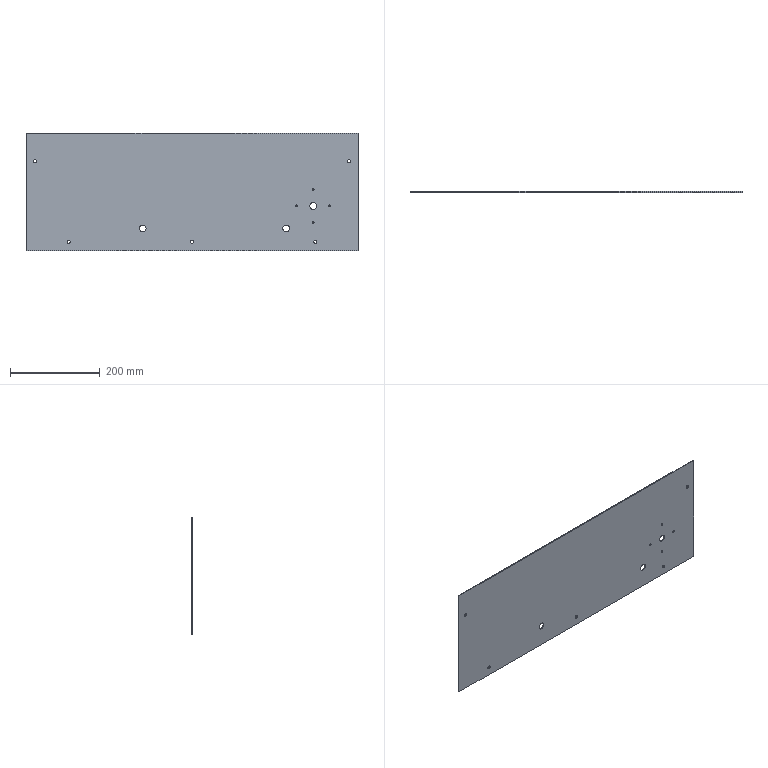Component | SolidWorks | 30-42A-1 | 1 solid | 30 faces | box 740 x 2 x 262 mm | volume 386204 mm3 | cylinder 24 | plane 6 | commonest cylinder face diameters 7 x10 4.2 x8 15 x6
build123d program:
from build123d import *

# Parameters (mm, degrees)
SKETCH1_W             = 740
SKETCH1_H             = 262
EXTRUDE1_DEPTH        = 2
SKETCH2_R             = 7.5
CUT_EXTRUDE1_DEPTH    = 10
SKETCH3_R             = 3.5
CUT_EXTRUDE2_DEPTH    = 10
M5_TAPPED_HOLE1_D     = 4.2
M5_TAPPED_HOLE1_DEPTH = 12.4
M5_TAPPED_HOLE1_TIP   = 1.262


with BuildPart() as part:
    # Sketch1 → Extrude1 (new body)
    with BuildSketch(Plane.XY):
        Rectangle(SKETCH1_W, SKETCH1_H)
    extrude(amount=EXTRUDE1_DEPTH)

    # Sketch2 → Cut-Extrude1 (cut)
    with BuildSketch(Plane.XY.offset(2)):
        with Locations((270, 31)):
            Circle(SKETCH2_R)
        with Locations((210, 81)):
            Circle(SKETCH2_R)
        with Locations((-110, 81)):
            Circle(SKETCH2_R)
    extrude(amount=-CUT_EXTRUDE1_DEPTH, mode=Mode.SUBTRACT)

    # Sketch3 → Cut-Extrude2 (cut)
    with BuildSketch(Plane.XY.offset(2)):
        with Locations((-275, 111)):
            Circle(SKETCH3_R)
        with Locations((0, 111)):
            Circle(SKETCH3_R)
        with Locations((-350, -69)):
            Circle(SKETCH3_R)
        with Locations((350, -69)):
            Circle(SKETCH3_R)
        with Locations((275, 111)):
            Circle(SKETCH3_R)
    extrude(amount=-CUT_EXTRUDE2_DEPTH, mode=Mode.SUBTRACT)

    # M5 Tapped Hole1
    with Locations(Plane.XY.offset(2)):
        with Locations((270, 67.5), (233.5, 31), (270, -5.5), (306.5, 31)):
            Hole(M5_TAPPED_HOLE1_D / 2, depth=M5_TAPPED_HOLE1_DEPTH)
            with Locations((0, 0, -(M5_TAPPED_HOLE1_DEPTH + M5_TAPPED_HOLE1_TIP / 2))):  # 118° drill point
                Cone(0, M5_TAPPED_HOLE1_D / 2, M5_TAPPED_HOLE1_TIP, mode=Mode.SUBTRACT)


solid = part.part

# Placed as in the assembly
solid = solid.moved(Location((-77.43, 712.155, -959), (-90, 0, 0)))
STEP:
#1=COLOUR_RGB('',0.7922,0.8196,0.9333);
#2=FILL_AREA_STYLE_COLOUR('',#1);
#3=FILL_AREA_STYLE('',(#2));
#4=SURFACE_STYLE_FILL_AREA(#3);
#5=SURFACE_SIDE_STYLE('',(#4));
#6=SURFACE_STYLE_USAGE(.BOTH.,#5);
#7=PRESENTATION_STYLE_ASSIGNMENT((#6));
#8=CARTESIAN_POINT('',(7.499,28.038,-40.413));
#9=VERTEX_POINT('',#8);
#10=CARTESIAN_POINT('',(7.664,28.038,-40.413));
#11=VERTEX_POINT('',#10);
#12=CARTESIAN_POINT('',(7.582,28.038,-40.413));
#13=DIRECTION('',(0.,1.,0.));
#14=DIRECTION('',(1.,0.,0.));
#15=AXIS2_PLACEMENT_3D('',#12,#13,#14);
#16=CIRCLE('',#15,0.08268);
#17=EDGE_CURVE('',#9,#11,#16,.T.);
#18=ORIENTED_EDGE('',*,*,#17,.F.);
#19=CARTESIAN_POINT('',(7.499,28.116,-40.413));
#20=VERTEX_POINT('',#19);
#21=CARTESIAN_POINT('',(7.499,28.116,-40.413));
#22=DIRECTION('',(0.,1.,0.));
#23=VECTOR('',#22,39.37);
#24=LINE('',#21,#23);
#25=EDGE_CURVE('',#9,#20,#24,.T.);
#26=ORIENTED_EDGE('',*,*,#25,.T.);
#27=CARTESIAN_POINT('',(7.664,28.116,-40.413));
#28=VERTEX_POINT('',#27);
#29=CARTESIAN_POINT('',(7.582,28.116,-40.413));
#30=DIRECTION('',(0.,1.,0.));
#31=DIRECTION('',(1.,0.,0.));
#32=AXIS2_PLACEMENT_3D('',#29,#30,#31);
#33=CIRCLE('',#32,0.08268);
#34=EDGE_CURVE('',#20,#28,#33,.T.);
#35=ORIENTED_EDGE('',*,*,#34,.T.);
#36=CARTESIAN_POINT('',(7.664,28.116,-40.413));
#37=DIRECTION('',(0.,1.,0.));
#38=VECTOR('',#37,39.37);
#39=LINE('',#36,#38);
#40=EDGE_CURVE('',#11,#28,#39,.T.);
#41=ORIENTED_EDGE('',*,*,#40,.F.);
#42=EDGE_LOOP('',(#18,#26,#35,#41));
#43=FACE_OUTER_BOUND('',#42,.T.);
#44=CARTESIAN_POINT('',(7.582,28.116,-40.413));
#45=DIRECTION('',(0.,1.,0.));
#46=DIRECTION('',(1.,0.,0.));
#47=AXIS2_PLACEMENT_3D('',#44,#45,#46);
#48=CYLINDRICAL_SURFACE('',#47,0.08268);
#49=ADVANCED_FACE('',(#43),#48,.F.);
#50=CARTESIAN_POINT('',(6.062,28.038,-38.976));
#51=VERTEX_POINT('',#50);
#52=CARTESIAN_POINT('',(6.227,28.038,-38.976));
#53=VERTEX_POINT('',#52);
#54=CARTESIAN_POINT('',(6.145,28.038,-38.976));
#55=DIRECTION('',(0.,1.,0.));
#56=DIRECTION('',(1.,0.,0.));
#57=AXIS2_PLACEMENT_3D('',#54,#55,#56);
#58=CIRCLE('',#57,0.08268);
#59=EDGE_CURVE('',#51,#53,#58,.T.);
#60=ORIENTED_EDGE('',*,*,#59,.F.);
#61=CARTESIAN_POINT('',(6.062,28.116,-38.976));
#62=VERTEX_POINT('',#61);
#63=CARTESIAN_POINT('',(6.062,28.116,-38.976));
#64=DIRECTION('',(0.,1.,0.));
#65=VECTOR('',#64,39.37);
#66=LINE('',#63,#65);
#67=EDGE_CURVE('',#51,#62,#66,.T.);
#68=ORIENTED_EDGE('',*,*,#67,.T.);
#69=CARTESIAN_POINT('',(6.227,28.116,-38.976));
#70=VERTEX_POINT('',#69);
#71=CARTESIAN_POINT('',(6.145,28.116,-38.976));
#72=DIRECTION('',(0.,1.,0.));
#73=DIRECTION('',(1.,0.,0.));
#74=AXIS2_PLACEMENT_3D('',#71,#72,#73);
#75=CIRCLE('',#74,0.08268);
#76=EDGE_CURVE('',#62,#70,#75,.T.);
#77=ORIENTED_EDGE('',*,*,#76,.T.);
#78=CARTESIAN_POINT('',(6.227,28.116,-38.976));
#79=DIRECTION('',(0.,1.,0.));
#80=VECTOR('',#79,39.37);
#81=LINE('',#78,#80);
#82=EDGE_CURVE('',#53,#70,#81,.T.);
#83=ORIENTED_EDGE('',*,*,#82,.F.);
#84=EDGE_LOOP('',(#60,#68,#77,#83));
#85=FACE_OUTER_BOUND('',#84,.T.);
#86=CARTESIAN_POINT('',(6.145,28.116,-38.976));
#87=DIRECTION('',(0.,1.,0.));
#88=DIRECTION('',(1.,0.,0.));
#89=AXIS2_PLACEMENT_3D('',#86,#87,#88);
#90=CYLINDRICAL_SURFACE('',#89,0.08268);
#91=ADVANCED_FACE('',(#85),#90,.F.);
#92=CARTESIAN_POINT('',(7.499,28.038,-37.539));
#93=VERTEX_POINT('',#92);
#94=CARTESIAN_POINT('',(7.664,28.038,-37.539));
#95=VERTEX_POINT('',#94);
#96=CARTESIAN_POINT('',(7.582,28.038,-37.539));
#97=DIRECTION('',(0.,1.,0.));
#98=DIRECTION('',(1.,0.,0.));
#99=AXIS2_PLACEMENT_3D('',#96,#97,#98);
#100=CIRCLE('',#99,0.08268);
#101=EDGE_CURVE('',#93,#95,#100,.T.);
#102=ORIENTED_EDGE('',*,*,#101,.F.);
#103=CARTESIAN_POINT('',(7.499,28.116,-37.539));
#104=VERTEX_POINT('',#103);
#105=CARTESIAN_POINT('',(7.499,28.116,-37.539));
#106=DIRECTION('',(0.,1.,0.));
#107=VECTOR('',#106,39.37);
#108=LINE('',#105,#107);
#109=EDGE_CURVE('',#93,#104,#108,.T.);
#110=ORIENTED_EDGE('',*,*,#109,.T.);
#111=CARTESIAN_POINT('',(7.664,28.116,-37.539));
#112=VERTEX_POINT('',#111);
#113=CARTESIAN_POINT('',(7.582,28.116,-37.539));
#114=DIRECTION('',(0.,1.,0.));
#115=DIRECTION('',(1.,0.,0.));
#116=AXIS2_PLACEMENT_3D('',#113,#114,#115);
#117=CIRCLE('',#116,0.08268);
#118=EDGE_CURVE('',#104,#112,#117,.T.);
#119=ORIENTED_EDGE('',*,*,#118,.T.);
#120=CARTESIAN_POINT('',(7.664,28.116,-37.539));
#121=DIRECTION('',(0.,1.,0.));
#122=VECTOR('',#121,39.37);
#123=LINE('',#120,#122);
#124=EDGE_CURVE('',#95,#112,#123,.T.);
#125=ORIENTED_EDGE('',*,*,#124,.F.);
#126=EDGE_LOOP('',(#102,#110,#119,#125));
#127=FACE_OUTER_BOUND('',#126,.T.);
#128=CARTESIAN_POINT('',(7.582,28.116,-37.539));
#129=DIRECTION('',(0.,1.,0.));
#130=DIRECTION('',(1.,0.,0.));
#131=AXIS2_PLACEMENT_3D('',#128,#129,#130);
#132=CYLINDRICAL_SURFACE('',#131,0.08268);
#133=ADVANCED_FACE('',(#127),#132,.F.);
#134=CARTESIAN_POINT('',(8.936,28.038,-38.976));
#135=VERTEX_POINT('',#134);
#136=CARTESIAN_POINT('',(9.101,28.038,-38.976));
#137=VERTEX_POINT('',#136);
#138=CARTESIAN_POINT('',(9.019,28.038,-38.976));
#139=DIRECTION('',(0.,1.,0.));
#140=DIRECTION('',(1.,0.,0.));
#141=AXIS2_PLACEMENT_3D('',#138,#139,#140);
#142=CIRCLE('',#141,0.08268);
#143=EDGE_CURVE('',#135,#137,#142,.T.);
#144=ORIENTED_EDGE('',*,*,#143,.F.);
#145=CARTESIAN_POINT('',(8.936,28.116,-38.976));
#146=VERTEX_POINT('',#145);
#147=CARTESIAN_POINT('',(8.936,28.116,-38.976));
#148=DIRECTION('',(0.,1.,0.));
#149=VECTOR('',#148,39.37);
#150=LINE('',#147,#149);
#151=EDGE_CURVE('',#135,#146,#150,.T.);
#152=ORIENTED_EDGE('',*,*,#151,.T.);
#153=CARTESIAN_POINT('',(9.101,28.116,-38.976));
#154=VERTEX_POINT('',#153);
#155=CARTESIAN_POINT('',(9.019,28.116,-38.976));
#156=DIRECTION('',(0.,1.,0.));
#157=DIRECTION('',(1.,0.,0.));
#158=AXIS2_PLACEMENT_3D('',#155,#156,#157);
#159=CIRCLE('',#158,0.08268);
#160=EDGE_CURVE('',#146,#154,#159,.T.);
#161=ORIENTED_EDGE('',*,*,#160,.T.);
#162=CARTESIAN_POINT('',(9.101,28.116,-38.976));
#163=DIRECTION('',(0.,1.,0.));
#164=VECTOR('',#163,39.37);
#165=LINE('',#162,#164);
#166=EDGE_CURVE('',#137,#154,#165,.T.);
#167=ORIENTED_EDGE('',*,*,#166,.F.);
#168=EDGE_LOOP('',(#144,#152,#161,#167));
#169=FACE_OUTER_BOUND('',#168,.T.);
#170=CARTESIAN_POINT('',(9.019,28.116,-38.976));
#171=DIRECTION('',(0.,1.,0.));
#172=DIRECTION('',(1.,0.,0.));
#173=AXIS2_PLACEMENT_3D('',#170,#171,#172);
#174=CYLINDRICAL_SURFACE('',#173,0.08268);
#175=ADVANCED_FACE('',(#169),#174,.F.);
#176=CARTESIAN_POINT('',(7.641,28.038,-42.126));
#177=VERTEX_POINT('',#176);
#178=CARTESIAN_POINT('',(7.916,28.038,-42.126));
#179=VERTEX_POINT('',#178);
#180=CARTESIAN_POINT('',(7.778,28.038,-42.126));
#181=DIRECTION('',(0.,1.,0.));
#182=DIRECTION('',(1.,0.,0.));
#183=AXIS2_PLACEMENT_3D('',#180,#181,#182);
#184=CIRCLE('',#183,0.1378);
#185=EDGE_CURVE('',#177,#179,#184,.T.);
#186=ORIENTED_EDGE('',*,*,#185,.F.);
#187=CARTESIAN_POINT('',(7.641,28.116,-42.126));
#188=VERTEX_POINT('',#187);
#189=CARTESIAN_POINT('',(7.641,27.723,-42.126));
#190=DIRECTION('',(0.,1.,0.));
#191=VECTOR('',#190,39.37);
#192=LINE('',#189,#191);
#193=EDGE_CURVE('',#177,#188,#192,.T.);
#194=ORIENTED_EDGE('',*,*,#193,.T.);
#195=CARTESIAN_POINT('',(7.916,28.116,-42.126));
#196=VERTEX_POINT('',#195);
#197=CARTESIAN_POINT('',(7.778,28.116,-42.126));
#198=DIRECTION('',(0.,1.,0.));
#199=DIRECTION('',(-1.,0.,0.));
#200=AXIS2_PLACEMENT_3D('',#197,#198,#199);
#201=CIRCLE('',#200,0.1378);
#202=EDGE_CURVE('',#188,#196,#201,.T.);
#203=ORIENTED_EDGE('',*,*,#202,.T.);
#204=CARTESIAN_POINT('',(7.916,27.723,-42.126));
#205=DIRECTION('',(0.,1.,0.));
#206=VECTOR('',#205,39.37);
#207=LINE('',#204,#206);
#208=EDGE_CURVE('',#179,#196,#207,.T.);
#209=ORIENTED_EDGE('',*,*,#208,.F.);
#210=EDGE_LOOP('',(#186,#194,#203,#209));
#211=FACE_OUTER_BOUND('',#210,.T.);
#212=CARTESIAN_POINT('',(7.778,27.723,-42.126));
#213=DIRECTION('',(0.,1.,0.));
#214=DIRECTION('',(1.,0.,0.));
#215=AXIS2_PLACEMENT_3D('',#212,#213,#214);
#216=CYLINDRICAL_SURFACE('',#215,0.1378);
#217=ADVANCED_FACE('',(#211),#216,.F.);
#218=CARTESIAN_POINT('',(10.593,28.038,-35.039));
#219=VERTEX_POINT('',#218);
#220=CARTESIAN_POINT('',(10.869,28.038,-35.039));
#221=VERTEX_POINT('',#220);
#222=CARTESIAN_POINT('',(10.731,28.038,-35.039));
#223=DIRECTION('',(0.,1.,0.));
#224=DIRECTION('',(1.,0.,0.));
#225=AXIS2_PLACEMENT_3D('',#222,#223,#224);
#226=CIRCLE('',#225,0.1378);
#227=EDGE_CURVE('',#219,#221,#226,.T.);
#228=ORIENTED_EDGE('',*,*,#227,.F.);
#229=CARTESIAN_POINT('',(10.593,28.116,-35.039));
#230=VERTEX_POINT('',#229);
#231=CARTESIAN_POINT('',(10.593,27.723,-35.039));
#232=DIRECTION('',(0.,1.,0.));
#233=VECTOR('',#232,39.37);
#234=LINE('',#231,#233);
#235=EDGE_CURVE('',#219,#230,#234,.T.);
#236=ORIENTED_EDGE('',*,*,#235,.T.);
#237=CARTESIAN_POINT('',(10.869,28.116,-35.039));
#238=VERTEX_POINT('',#237);
#239=CARTESIAN_POINT('',(10.731,28.116,-35.039));
#240=DIRECTION('',(0.,1.,0.));
#241=DIRECTION('',(-1.,0.,0.));
#242=AXIS2_PLACEMENT_3D('',#239,#240,#241);
#243=CIRCLE('',#242,0.1378);
#244=EDGE_CURVE('',#230,#238,#243,.T.);
#245=ORIENTED_EDGE('',*,*,#244,.T.);
#246=CARTESIAN_POINT('',(10.869,27.723,-35.039));
#247=DIRECTION('',(0.,1.,0.));
#248=VECTOR('',#247,39.37);
#249=LINE('',#246,#248);
#250=EDGE_CURVE('',#221,#238,#249,.T.);
#251=ORIENTED_EDGE('',*,*,#250,.F.);
#252=EDGE_LOOP('',(#228,#236,#245,#251));
#253=FACE_OUTER_BOUND('',#252,.T.);
#254=CARTESIAN_POINT('',(10.731,27.723,-35.039));
#255=DIRECTION('',(0.,1.,0.));
#256=DIRECTION('',(1.,0.,0.));
#257=AXIS2_PLACEMENT_3D('',#254,#255,#256);
#258=CYLINDRICAL_SURFACE('',#257,0.1378);
#259=ADVANCED_FACE('',(#253),#258,.F.);
#260=CARTESIAN_POINT('',(-16.966,28.038,-35.039));
#261=VERTEX_POINT('',#260);
#262=CARTESIAN_POINT('',(-16.69,28.038,-35.039));
#263=VERTEX_POINT('',#262);
#264=CARTESIAN_POINT('',(-16.828,28.038,-35.039));
#265=DIRECTION('',(0.,1.,0.));
#266=DIRECTION('',(1.,0.,0.));
#267=AXIS2_PLACEMENT_3D('',#264,#265,#266);
#268=CIRCLE('',#267,0.1378);
#269=EDGE_CURVE('',#261,#263,#268,.T.);
#270=ORIENTED_EDGE('',*,*,#269,.F.);
#271=CARTESIAN_POINT('',(-16.966,28.116,-35.039));
#272=VERTEX_POINT('',#271);
#273=CARTESIAN_POINT('',(-16.966,27.723,-35.039));
#274=DIRECTION('',(0.,1.,0.));
#275=VECTOR('',#274,39.37);
#276=LINE('',#273,#275);
#277=EDGE_CURVE('',#261,#272,#276,.T.);
#278=ORIENTED_EDGE('',*,*,#277,.T.);
#279=CARTESIAN_POINT('',(-16.69,28.116,-35.039));
#280=VERTEX_POINT('',#279);
#281=CARTESIAN_POINT('',(-16.828,28.116,-35.039));
#282=DIRECTION('',(0.,1.,0.));
#283=DIRECTION('',(1.,0.,0.));
#284=AXIS2_PLACEMENT_3D('',#281,#282,#283);
#285=CIRCLE('',#284,0.1378);
#286=EDGE_CURVE('',#272,#280,#285,.T.);
#287=ORIENTED_EDGE('',*,*,#286,.T.);
#288=CARTESIAN_POINT('',(-16.69,27.723,-35.039));
#289=DIRECTION('',(0.,1.,0.));
#290=VECTOR('',#289,39.37);
#291=LINE('',#288,#290);
#292=EDGE_CURVE('',#263,#280,#291,.T.);
#293=ORIENTED_EDGE('',*,*,#292,.F.);
#294=EDGE_LOOP('',(#270,#278,#287,#293));
#295=FACE_OUTER_BOUND('',#294,.T.);
#296=CARTESIAN_POINT('',(-16.828,27.723,-35.039));
#297=DIRECTION('',(0.,1.,0.));
#298=DIRECTION('',(1.,0.,0.));
#299=AXIS2_PLACEMENT_3D('',#296,#297,#298);
#300=CYLINDRICAL_SURFACE('',#299,0.1378);
#301=ADVANCED_FACE('',(#295),#300,.F.);
#302=CARTESIAN_POINT('',(-3.186,28.038,-42.126));
#303=VERTEX_POINT('',#302);
#304=CARTESIAN_POINT('',(-2.911,28.038,-42.126));
#305=VERTEX_POINT('',#304);
#306=CARTESIAN_POINT('',(-3.048,28.038,-42.126));
#307=DIRECTION('',(0.,1.,0.));
#308=DIRECTION('',(1.,0.,0.));
#309=AXIS2_PLACEMENT_3D('',#306,#307,#308);
#310=CIRCLE('',#309,0.1378);
#311=EDGE_CURVE('',#303,#305,#310,.T.);
#312=ORIENTED_EDGE('',*,*,#311,.F.);
#313=CARTESIAN_POINT('',(-3.186,28.116,-42.126));
#314=VERTEX_POINT('',#313);
#315=CARTESIAN_POINT('',(-3.186,27.723,-42.126));
#316=DIRECTION('',(0.,1.,0.));
#317=VECTOR('',#316,39.37);
#318=LINE('',#315,#317);
#319=EDGE_CURVE('',#303,#314,#318,.T.);
#320=ORIENTED_EDGE('',*,*,#319,.T.);
#321=CARTESIAN_POINT('',(-2.911,28.116,-42.126));
#322=VERTEX_POINT('',#321);
#323=CARTESIAN_POINT('',(-3.048,28.116,-42.126));
#324=DIRECTION('',(0.,1.,0.));
#325=DIRECTION('',(1.,0.,0.));
#326=AXIS2_PLACEMENT_3D('',#323,#324,#325);
#327=CIRCLE('',#326,0.1378);
#328=EDGE_CURVE('',#314,#322,#327,.T.);
#329=ORIENTED_EDGE('',*,*,#328,.T.);
#330=CARTESIAN_POINT('',(-2.911,27.723,-42.126));
#331=DIRECTION('',(0.,1.,0.));
#332=VECTOR('',#331,39.37);
#333=LINE('',#330,#332);
#334=EDGE_CURVE('',#305,#322,#333,.T.);
#335=ORIENTED_EDGE('',*,*,#334,.F.);
#336=EDGE_LOOP('',(#312,#320,#329,#335));
#337=FACE_OUTER_BOUND('',#336,.T.);
#338=CARTESIAN_POINT('',(-3.048,27.723,-42.126));
#339=DIRECTION('',(0.,1.,0.));
#340=DIRECTION('',(1.,0.,0.));
#341=AXIS2_PLACEMENT_3D('',#338,#339,#340);
#342=CYLINDRICAL_SURFACE('',#341,0.1378);
#343=ADVANCED_FACE('',(#337),#342,.F.);
#344=CARTESIAN_POINT('',(-14.013,28.038,-42.126));
#345=VERTEX_POINT('',#344);
#346=CARTESIAN_POINT('',(-13.737,28.038,-42.126));
#347=VERTEX_POINT('',#346);
#348=CARTESIAN_POINT('',(-13.875,28.038,-42.126));
#349=DIRECTION('',(0.,1.,0.));
#350=DIRECTION('',(1.,0.,0.));
#351=AXIS2_PLACEMENT_3D('',#348,#349,#350);
#352=CIRCLE('',#351,0.1378);
#353=EDGE_CURVE('',#345,#347,#352,.T.);
#354=ORIENTED_EDGE('',*,*,#353,.F.);
#355=CARTESIAN_POINT('',(-14.013,28.116,-42.126));
#356=VERTEX_POINT('',#355);
#357=CARTESIAN_POINT('',(-14.013,27.723,-42.126));
#358=DIRECTION('',(0.,1.,0.));
#359=VECTOR('',#358,39.37);
#360=LINE('',#357,#359);
#361=EDGE_CURVE('',#345,#356,#360,.T.);
#362=ORIENTED_EDGE('',*,*,#361,.T.);
#363=CARTESIAN_POINT('',(-13.737,28.116,-42.126));
#364=VERTEX_POINT('',#363);
#365=CARTESIAN_POINT('',(-13.875,28.116,-42.126));
#366=DIRECTION('',(0.,1.,0.));
#367=DIRECTION('',(1.,0.,0.));
#368=AXIS2_PLACEMENT_3D('',#365,#366,#367);
#369=CIRCLE('',#368,0.1378);
#370=EDGE_CURVE('',#356,#364,#369,.T.);
#371=ORIENTED_EDGE('',*,*,#370,.T.);
#372=CARTESIAN_POINT('',(-13.737,27.723,-42.126));
#373=DIRECTION('',(0.,1.,0.));
#374=VECTOR('',#373,39.37);
#375=LINE('',#372,#374);
#376=EDGE_CURVE('',#347,#364,#375,.T.);
#377=ORIENTED_EDGE('',*,*,#376,.F.);
#378=EDGE_LOOP('',(#354,#362,#371,#377));
#379=FACE_OUTER_BOUND('',#378,.T.);
#380=CARTESIAN_POINT('',(-13.875,27.723,-42.126));
#381=DIRECTION('',(0.,1.,0.));
#382=DIRECTION('',(1.,0.,0.));
#383=AXIS2_PLACEMENT_3D('',#380,#381,#382);
#384=CYLINDRICAL_SURFACE('',#383,0.1378);
#385=ADVANCED_FACE('',(#379),#384,.F.);
#386=CARTESIAN_POINT('',(-7.674,28.038,-40.945));
#387=VERTEX_POINT('',#386);
#388=CARTESIAN_POINT('',(-7.084,28.038,-40.945));
#389=VERTEX_POINT('',#388);
#390=CARTESIAN_POINT('',(-7.379,28.038,-40.945));
#391=DIRECTION('',(0.,1.,0.));
#392=DIRECTION('',(1.,0.,0.));
#393=AXIS2_PLACEMENT_3D('',#390,#391,#392);
#394=CIRCLE('',#393,0.2953);
#395=EDGE_CURVE('',#387,#389,#394,.T.);
#396=ORIENTED_EDGE('',*,*,#395,.F.);
#397=CARTESIAN_POINT('',(-7.674,28.116,-40.945));
#398=VERTEX_POINT('',#397);
#399=CARTESIAN_POINT('',(-7.674,27.723,-40.945));
#400=DIRECTION('',(0.,1.,0.));
#401=VECTOR('',#400,39.37);
#402=LINE('',#399,#401);
#403=EDGE_CURVE('',#387,#398,#402,.T.);
#404=ORIENTED_EDGE('',*,*,#403,.T.);
#405=CARTESIAN_POINT('',(-7.084,28.116,-40.945));
#406=VERTEX_POINT('',#405);
#407=CARTESIAN_POINT('',(-7.379,28.116,-40.945));
#408=DIRECTION('',(0.,1.,0.));
#409=DIRECTION('',(1.,0.,0.));
#410=AXIS2_PLACEMENT_3D('',#407,#408,#409);
#411=CIRCLE('',#410,0.2953);
#412=EDGE_CURVE('',#398,#406,#411,.T.);
#413=ORIENTED_EDGE('',*,*,#412,.T.);
#414=CARTESIAN_POINT('',(-7.084,27.723,-40.945));
#415=DIRECTION('',(0.,1.,0.));
#416=VECTOR('',#415,39.37);
#417=LINE('',#414,#416);
#418=EDGE_CURVE('',#389,#406,#417,.T.);
#419=ORIENTED_EDGE('',*,*,#418,.F.);
#420=EDGE_LOOP('',(#396,#404,#413,#419));
#421=FACE_OUTER_BOUND('',#420,.T.);
#422=CARTESIAN_POINT('',(-7.379,27.723,-40.945));
#423=DIRECTION('',(0.,1.,0.));
#424=DIRECTION('',(1.,0.,0.));
#425=AXIS2_PLACEMENT_3D('',#422,#423,#424);
#426=CYLINDRICAL_SURFACE('',#425,0.2953);
#427=ADVANCED_FACE('',(#421),#426,.F.);
#428=CARTESIAN_POINT('',(4.924,28.038,-40.945));
#429=VERTEX_POINT('',#428);
#430=CARTESIAN_POINT('',(5.515,28.038,-40.945));
#431=VERTEX_POINT('',#430);
#432=CARTESIAN_POINT('',(5.219,28.038,-40.945));
#433=DIRECTION('',(0.,1.,0.));
#434=DIRECTION('',(1.,0.,0.));
#435=AXIS2_PLACEMENT_3D('',#432,#433,#434);
#436=CIRCLE('',#435,0.2953);
#437=EDGE_CURVE('',#429,#431,#436,.T.);
#438=ORIENTED_EDGE('',*,*,#437,.F.);
#439=CARTESIAN_POINT('',(4.924,28.116,-40.945));
#440=VERTEX_POINT('',#439);
#441=CARTESIAN_POINT('',(4.924,27.723,-40.945));
#442=DIRECTION('',(0.,1.,0.));
#443=VECTOR('',#442,39.37);
#444=LINE('',#441,#443);
#445=EDGE_CURVE('',#429,#440,#444,.T.);
#446=ORIENTED_EDGE('',*,*,#445,.T.);
#447=CARTESIAN_POINT('',(5.515,28.116,-40.945));
#448=VERTEX_POINT('',#447);
#449=CARTESIAN_POINT('',(5.219,28.116,-40.945));
#450=DIRECTION('',(0.,1.,0.));
#451=DIRECTION('',(1.,0.,0.));
#452=AXIS2_PLACEMENT_3D('',#449,#450,#451);
#453=CIRCLE('',#452,0.2953);
#454=EDGE_CURVE('',#440,#448,#453,.T.);
#455=ORIENTED_EDGE('',*,*,#454,.T.);
#456=CARTESIAN_POINT('',(5.515,27.723,-40.945));
#457=DIRECTION('',(0.,1.,0.));
#458=VECTOR('',#457,39.37);
#459=LINE('',#456,#458);
#460=EDGE_CURVE('',#431,#448,#459,.T.);
#461=ORIENTED_EDGE('',*,*,#460,.F.);
#462=EDGE_LOOP('',(#438,#446,#455,#461));
#463=FACE_OUTER_BOUND('',#462,.T.);
#464=CARTESIAN_POINT('',(5.219,27.723,-40.945));
#465=DIRECTION('',(0.,1.,0.));
#466=DIRECTION('',(1.,0.,0.));
#467=AXIS2_PLACEMENT_3D('',#464,#465,#466);
#468=CYLINDRICAL_SURFACE('',#467,0.2953);
#469=ADVANCED_FACE('',(#463),#468,.F.);
#470=CARTESIAN_POINT('',(7.286,28.038,-38.976));
#471=VERTEX_POINT('',#470);
#472=CARTESIAN_POINT('',(7.877,28.038,-38.976));
#473=VERTEX_POINT('',#472);
#474=CARTESIAN_POINT('',(7.582,28.038,-38.976));
#475=DIRECTION('',(0.,1.,0.));
#476=DIRECTION('',(1.,0.,0.));
#477=AXIS2_PLACEMENT_3D('',#474,#475,#476);
#478=CIRCLE('',#477,0.2953);
#479=EDGE_CURVE('',#471,#473,#478,.T.);
#480=ORIENTED_EDGE('',*,*,#479,.F.);
#481=CARTESIAN_POINT('',(7.286,28.116,-38.976));
#482=VERTEX_POINT('',#481);
#483=CARTESIAN_POINT('',(7.286,27.723,-38.976));
#484=DIRECTION('',(0.,1.,0.));
#485=VECTOR('',#484,39.37);
#486=LINE('',#483,#485);
#487=EDGE_CURVE('',#471,#482,#486,.T.);
#488=ORIENTED_EDGE('',*,*,#487,.T.);
#489=CARTESIAN_POINT('',(7.877,28.116,-38.976));
#490=VERTEX_POINT('',#489);
#491=CARTESIAN_POINT('',(7.582,28.116,-38.976));
#492=DIRECTION('',(0.,1.,0.));
#493=DIRECTION('',(1.,0.,0.));
#494=AXIS2_PLACEMENT_3D('',#491,#492,#493);
#495=CIRCLE('',#494,0.2953);
#496=EDGE_CURVE('',#482,#490,#495,.T.);
#497=ORIENTED_EDGE('',*,*,#496,.T.);
#498=CARTESIAN_POINT('',(7.877,27.723,-38.976));
#499=DIRECTION('',(0.,1.,0.));
#500=VECTOR('',#499,39.37);
#501=LINE('',#498,#500);
#502=EDGE_CURVE('',#473,#490,#501,.T.);
#503=ORIENTED_EDGE('',*,*,#502,.F.);
#504=EDGE_LOOP('',(#480,#488,#497,#503));
#505=FACE_OUTER_BOUND('',#504,.T.);
#506=CARTESIAN_POINT('',(7.582,27.723,-38.976));
#507=DIRECTION('',(0.,1.,0.));
#508=DIRECTION('',(1.,0.,0.));
#509=AXIS2_PLACEMENT_3D('',#506,#507,#508);
#510=CYLINDRICAL_SURFACE('',#509,0.2953);
#511=ADVANCED_FACE('',(#505),#510,.F.);
#512=CARTESIAN_POINT('',(-17.615,28.038,-42.913));
#513=VERTEX_POINT('',#512);
#514=CARTESIAN_POINT('',(-17.615,28.038,-32.598));
#515=VERTEX_POINT('',#514);
#516=CARTESIAN_POINT('',(-17.615,28.038,-42.913));
#517=DIRECTION('',(0.,-0.,1.));
#518=VECTOR('',#517,39.37);
#519=LINE('',#516,#518);
#520=EDGE_CURVE('',#513,#515,#519,.T.);
#521=ORIENTED_EDGE('',*,*,#520,.T.);
#522=CARTESIAN_POINT('',(-17.615,28.116,-32.598));
#523=VERTEX_POINT('',#522);
#524=CARTESIAN_POINT('',(-17.615,28.116,-32.598));
#525=DIRECTION('',(-0.,-1.,-0.));
#526=VECTOR('',#525,39.37);
#527=LINE('',#524,#526);
#528=EDGE_CURVE('',#523,#515,#527,.T.);
#529=ORIENTED_EDGE('',*,*,#528,.F.);
#530=CARTESIAN_POINT('',(-17.615,28.116,-42.913));
#531=VERTEX_POINT('',#530);
#532=CARTESIAN_POINT('',(-17.615,28.116,-42.913));
#533=DIRECTION('',(0.,-0.,1.));
#534=VECTOR('',#533,39.37);
#535=LINE('',#532,#534);
#536=EDGE_CURVE('',#531,#523,#535,.T.);
#537=ORIENTED_EDGE('',*,*,#536,.F.);
#538=CARTESIAN_POINT('',(-17.615,28.116,-42.913));
#539=DIRECTION('',(-0.,-1.,-0.));
#540=VECTOR('',#539,39.37);
#541=LINE('',#538,#540);
#542=EDGE_CURVE('',#531,#513,#541,.T.);
#543=ORIENTED_EDGE('',*,*,#542,.T.);
#544=EDGE_LOOP('',(#521,#529,#537,#543));
#545=FACE_OUTER_BOUND('',#544,.T.);
#546=CARTESIAN_POINT('',(-17.615,28.116,-42.913));
#547=DIRECTION('',(1.,0.,-0.));
#548=DIRECTION('',(-0.,0.,-1.));
#549=AXIS2_PLACEMENT_3D('',#546,#547,#548);
#550=PLANE('',#549);
#551=ADVANCED_FACE('',(#545),#550,.F.);
#552=CARTESIAN_POINT('',(11.519,28.038,-32.598));
#553=VERTEX_POINT('',#552);
#554=CARTESIAN_POINT('',(-17.615,28.038,-32.598));
#555=DIRECTION('',(1.,0.,0.));
#556=VECTOR('',#555,39.37);
#557=LINE('',#554,#556);
#558=EDGE_CURVE('',#515,#553,#557,.T.);
#559=ORIENTED_EDGE('',*,*,#558,.T.);
#560=CARTESIAN_POINT('',(11.519,28.116,-32.598));
#561=VERTEX_POINT('',#560);
#562=CARTESIAN_POINT('',(11.519,28.116,-32.598));
#563=DIRECTION('',(-0.,-1.,-0.));
#564=VECTOR('',#563,39.37);
#565=LINE('',#562,#564);
#566=EDGE_CURVE('',#561,#553,#565,.T.);
#567=ORIENTED_EDGE('',*,*,#566,.F.);
#568=CARTESIAN_POINT('',(-17.615,28.116,-32.598));
#569=DIRECTION('',(1.,0.,0.));
#570=VECTOR('',#569,39.37);
#571=LINE('',#568,#570);
#572=EDGE_CURVE('',#523,#561,#571,.T.);
#573=ORIENTED_EDGE('',*,*,#572,.F.);
#574=ORIENTED_EDGE('',*,*,#528,.T.);
#575=EDGE_LOOP('',(#559,#567,#573,#574));
#576=FACE_OUTER_BOUND('',#575,.T.);
#577=CARTESIAN_POINT('',(-17.615,28.116,-32.598));
#578=DIRECTION('',(0.,0.,-1.));
#579=DIRECTION('',(0.,1.,0.));
#580=AXIS2_PLACEMENT_3D('',#577,#578,#579);
#581=PLANE('',#580);
#582=ADVANCED_FACE('',(#576),#581,.F.);
#583=CARTESIAN_POINT('',(11.519,28.038,-42.913));
#584=VERTEX_POINT('',#583);
#585=CARTESIAN_POINT('',(11.519,28.038,-42.913));
#586=DIRECTION('',(-0.,0.,-1.));
#587=VECTOR('',#586,39.37);
#588=LINE('',#585,#587);
#589=EDGE_CURVE('',#553,#584,#588,.T.);
#590=ORIENTED_EDGE('',*,*,#589,.T.);
#591=CARTESIAN_POINT('',(11.519,28.116,-42.913));
#592=VERTEX_POINT('',#591);
#593=CARTESIAN_POINT('',(11.519,28.116,-42.913));
#594=DIRECTION('',(-0.,-1.,-0.));
#595=VECTOR('',#594,39.37);
#596=LINE('',#593,#595);
#597=EDGE_CURVE('',#592,#584,#596,.T.);
#598=ORIENTED_EDGE('',*,*,#597,.F.);
#599=CARTESIAN_POINT('',(11.519,28.116,-42.913));
#600=DIRECTION('',(-0.,0.,-1.));
#601=VECTOR('',#600,39.37);
#602=LINE('',#599,#601);
#603=EDGE_CURVE('',#561,#592,#602,.T.);
#604=ORIENTED_EDGE('',*,*,#603,.F.);
#605=ORIENTED_EDGE('',*,*,#566,.T.);
#606=EDGE_LOOP('',(#590,#598,#604,#605));
#607=FACE_OUTER_BOUND('',#606,.T.);
#608=CARTESIAN_POINT('',(11.519,28.116,-42.913));
#609=DIRECTION('',(-1.,-0.,0.));
#610=DIRECTION('',(0.,-0.,1.));
#611=AXIS2_PLACEMENT_3D('',#608,#609,#610);
#612=PLANE('',#611);
#613=ADVANCED_FACE('',(#607),#612,.F.);
#614=CARTESIAN_POINT('',(-17.615,28.038,-42.913));
#615=DIRECTION('',(-1.,0.,-0.));
#616=VECTOR('',#615,39.37);
#617=LINE('',#614,#616);
#618=EDGE_CURVE('',#584,#513,#617,.T.);
#619=ORIENTED_EDGE('',*,*,#618,.T.);
#620=ORIENTED_EDGE('',*,*,#542,.F.);
#621=CARTESIAN_POINT('',(-17.615,28.116,-42.913));
#622=DIRECTION('',(-1.,0.,-0.));
#623=VECTOR('',#622,39.37);
#624=LINE('',#621,#623);
#625=EDGE_CURVE('',#592,#531,#624,.T.);
#626=ORIENTED_EDGE('',*,*,#625,.F.);
#627=ORIENTED_EDGE('',*,*,#597,.T.);
#628=EDGE_LOOP('',(#619,#620,#626,#627));
#629=FACE_OUTER_BOUND('',#628,.T.);
#630=CARTESIAN_POINT('',(-17.615,28.116,-42.913));
#631=DIRECTION('',(-0.,-0.,1.));
#632=DIRECTION('',(-0.,-1.,-0.));
#633=AXIS2_PLACEMENT_3D('',#630,#631,#632);
#634=PLANE('',#633);
#635=ADVANCED_FACE('',(#629),#634,.F.);
#636=CARTESIAN_POINT('',(7.582,28.116,-40.413));
#637=DIRECTION('',(0.,1.,0.));
#638=DIRECTION('',(1.,0.,0.));
#639=AXIS2_PLACEMENT_3D('',#636,#637,#638);
#640=CIRCLE('',#639,0.08268);
#641=EDGE_CURVE('',#28,#20,#640,.T.);
#642=ORIENTED_EDGE('',*,*,#641,.F.);
#643=ORIENTED_EDGE('',*,*,#34,.F.);
#644=EDGE_LOOP('',(#642,#643));
#645=FACE_BOUND('',#644,.T.);
#646=CARTESIAN_POINT('',(6.145,28.116,-38.976));
#647=DIRECTION('',(0.,1.,0.));
#648=DIRECTION('',(1.,0.,0.));
#649=AXIS2_PLACEMENT_3D('',#646,#647,#648);
#650=CIRCLE('',#649,0.08268);
#651=EDGE_CURVE('',#70,#62,#650,.T.);
#652=ORIENTED_EDGE('',*,*,#651,.F.);
#653=ORIENTED_EDGE('',*,*,#76,.F.);
#654=EDGE_LOOP('',(#652,#653));
#655=FACE_BOUND('',#654,.T.);
#656=CARTESIAN_POINT('',(7.582,28.116,-37.539));
#657=DIRECTION('',(0.,1.,0.));
#658=DIRECTION('',(1.,0.,0.));
#659=AXIS2_PLACEMENT_3D('',#656,#657,#658);
#660=CIRCLE('',#659,0.08268);
#661=EDGE_CURVE('',#112,#104,#660,.T.);
#662=ORIENTED_EDGE('',*,*,#661,.F.);
#663=ORIENTED_EDGE('',*,*,#118,.F.);
#664=EDGE_LOOP('',(#662,#663));
#665=FACE_BOUND('',#664,.T.);
#666=CARTESIAN_POINT('',(9.019,28.116,-38.976));
#667=DIRECTION('',(0.,1.,0.));
#668=DIRECTION('',(1.,0.,0.));
#669=AXIS2_PLACEMENT_3D('',#666,#667,#668);
#670=CIRCLE('',#669,0.08268);
#671=EDGE_CURVE('',#154,#146,#670,.T.);
#672=ORIENTED_EDGE('',*,*,#671,.F.);
#673=ORIENTED_EDGE('',*,*,#160,.F.);
#674=EDGE_LOOP('',(#672,#673));
#675=FACE_BOUND('',#674,.T.);
#676=CARTESIAN_POINT('',(7.778,28.116,-42.126));
#677=DIRECTION('',(0.,1.,0.));
#678=DIRECTION('',(-1.,0.,0.));
#679=AXIS2_PLACEMENT_3D('',#676,#677,#678);
#680=CIRCLE('',#679,0.1378);
#681=EDGE_CURVE('',#196,#188,#680,.T.);
#682=ORIENTED_EDGE('',*,*,#681,.F.);
#683=ORIENTED_EDGE('',*,*,#202,.F.);
#684=EDGE_LOOP('',(#682,#683));
#685=FACE_BOUND('',#684,.T.);
#686=CARTESIAN_POINT('',(10.731,28.116,-35.039));
#687=DIRECTION('',(0.,1.,0.));
#688=DIRECTION('',(-1.,0.,0.));
#689=AXIS2_PLACEMENT_3D('',#686,#687,#688);
#690=CIRCLE('',#689,0.1378);
#691=EDGE_CURVE('',#238,#230,#690,.T.);
#692=ORIENTED_EDGE('',*,*,#691,.F.);
#693=ORIENTED_EDGE('',*,*,#244,.F.);
#694=EDGE_LOOP('',(#692,#693));
#695=FACE_BOUND('',#694,.T.);
#696=CARTESIAN_POINT('',(-16.828,28.116,-35.039));
#697=DIRECTION('',(0.,1.,0.));
#698=DIRECTION('',(1.,0.,0.));
#699=AXIS2_PLACEMENT_3D('',#696,#697,#698);
#700=CIRCLE('',#699,0.1378);
#701=EDGE_CURVE('',#280,#272,#700,.T.);
#702=ORIENTED_EDGE('',*,*,#701,.F.);
#703=ORIENTED_EDGE('',*,*,#286,.F.);
#704=EDGE_LOOP('',(#702,#703));
#705=FACE_BOUND('',#704,.T.);
#706=CARTESIAN_POINT('',(-3.048,28.116,-42.126));
#707=DIRECTION('',(0.,1.,0.));
#708=DIRECTION('',(1.,0.,0.));
#709=AXIS2_PLACEMENT_3D('',#706,#707,#708);
#710=CIRCLE('',#709,0.1378);
#711=EDGE_CURVE('',#322,#314,#710,.T.);
#712=ORIENTED_EDGE('',*,*,#711,.F.);
#713=ORIENTED_EDGE('',*,*,#328,.F.);
#714=EDGE_LOOP('',(#712,#713));
#715=FACE_BOUND('',#714,.T.);
#716=CARTESIAN_POINT('',(-13.875,28.116,-42.126));
#717=DIRECTION('',(0.,1.,0.));
#718=DIRECTION('',(1.,0.,0.));
#719=AXIS2_PLACEMENT_3D('',#716,#717,#718);
#720=CIRCLE('',#719,0.1378);
#721=EDGE_CURVE('',#364,#356,#720,.T.);
#722=ORIENTED_EDGE('',*,*,#721,.F.);
#723=ORIENTED_EDGE('',*,*,#370,.F.);
#724=EDGE_LOOP('',(#722,#723));
#725=FACE_BOUND('',#724,.T.);
#726=CARTESIAN_POINT('',(-7.379,28.116,-40.945));
#727=DIRECTION('',(0.,1.,0.));
#728=DIRECTION('',(1.,0.,0.));
#729=AXIS2_PLACEMENT_3D('',#726,#727,#728);
#730=CIRCLE('',#729,0.2953);
#731=EDGE_CURVE('',#406,#398,#730,.T.);
#732=ORIENTED_EDGE('',*,*,#731,.F.);
#733=ORIENTED_EDGE('',*,*,#412,.F.);
#734=EDGE_LOOP('',(#732,#733));
#735=FACE_BOUND('',#734,.T.);
#736=CARTESIAN_POINT('',(5.219,28.116,-40.945));
#737=DIRECTION('',(0.,1.,0.));
#738=DIRECTION('',(1.,0.,0.));
#739=AXIS2_PLACEMENT_3D('',#736,#737,#738);
#740=CIRCLE('',#739,0.2953);
#741=EDGE_CURVE('',#448,#440,#740,.T.);
#742=ORIENTED_EDGE('',*,*,#741,.F.);
#743=ORIENTED_EDGE('',*,*,#454,.F.);
#744=EDGE_LOOP('',(#742,#743));
#745=FACE_BOUND('',#744,.T.);
#746=CARTESIAN_POINT('',(7.582,28.116,-38.976));
#747=DIRECTION('',(0.,1.,0.));
#748=DIRECTION('',(1.,0.,0.));
#749=AXIS2_PLACEMENT_3D('',#746,#747,#748);
#750=CIRCLE('',#749,0.2953);
#751=EDGE_CURVE('',#490,#482,#750,.T.);
#752=ORIENTED_EDGE('',*,*,#751,.F.);
#753=ORIENTED_EDGE('',*,*,#496,.F.);
#754=EDGE_LOOP('',(#752,#753));
#755=FACE_BOUND('',#754,.T.);
#756=ORIENTED_EDGE('',*,*,#536,.T.);
#757=ORIENTED_EDGE('',*,*,#572,.T.);
#758=ORIENTED_EDGE('',*,*,#603,.T.);
#759=ORIENTED_EDGE('',*,*,#625,.T.);
#760=EDGE_LOOP('',(#756,#757,#758,#759));
#761=FACE_OUTER_BOUND('',#760,.T.);
#762=CARTESIAN_POINT('',(-17.615,28.116,-32.598));
#763=DIRECTION('',(-0.,1.,0.));
#764=DIRECTION('',(1.,0.,0.));
#765=AXIS2_PLACEMENT_3D('',#762,#763,#764);
#766=PLANE('',#765);
#767=ADVANCED_FACE('',(#645,#655,#665,#675,#685,#695,#705,#715,#725,#735,#745,#755,#761),#766,.T.);
#768=CARTESIAN_POINT('',(7.582,28.038,-40.413));
#769=DIRECTION('',(0.,1.,0.));
#770=DIRECTION('',(1.,0.,0.));
#771=AXIS2_PLACEMENT_3D('',#768,#769,#770);
#772=CIRCLE('',#771,0.08268);
#773=EDGE_CURVE('',#11,#9,#772,.T.);
#774=ORIENTED_EDGE('',*,*,#773,.T.);
#775=ORIENTED_EDGE('',*,*,#17,.T.);
#776=EDGE_LOOP('',(#774,#775));
#777=FACE_BOUND('',#776,.T.);
#778=CARTESIAN_POINT('',(6.145,28.038,-38.976));
#779=DIRECTION('',(0.,1.,0.));
#780=DIRECTION('',(1.,0.,0.));
#781=AXIS2_PLACEMENT_3D('',#778,#779,#780);
#782=CIRCLE('',#781,0.08268);
#783=EDGE_CURVE('',#53,#51,#782,.T.);
#784=ORIENTED_EDGE('',*,*,#783,.T.);
#785=ORIENTED_EDGE('',*,*,#59,.T.);
#786=EDGE_LOOP('',(#784,#785));
#787=FACE_BOUND('',#786,.T.);
#788=CARTESIAN_POINT('',(7.582,28.038,-37.539));
#789=DIRECTION('',(0.,1.,0.));
#790=DIRECTION('',(1.,0.,0.));
#791=AXIS2_PLACEMENT_3D('',#788,#789,#790);
#792=CIRCLE('',#791,0.08268);
#793=EDGE_CURVE('',#95,#93,#792,.T.);
#794=ORIENTED_EDGE('',*,*,#793,.T.);
#795=ORIENTED_EDGE('',*,*,#101,.T.);
#796=EDGE_LOOP('',(#794,#795));
#797=FACE_BOUND('',#796,.T.);
#798=CARTESIAN_POINT('',(9.019,28.038,-38.976));
#799=DIRECTION('',(0.,1.,0.));
#800=DIRECTION('',(1.,0.,0.));
#801=AXIS2_PLACEMENT_3D('',#798,#799,#800);
#802=CIRCLE('',#801,0.08268);
#803=EDGE_CURVE('',#137,#135,#802,.T.);
#804=ORIENTED_EDGE('',*,*,#803,.T.);
#805=ORIENTED_EDGE('',*,*,#143,.T.);
#806=EDGE_LOOP('',(#804,#805));
#807=FACE_BOUND('',#806,.T.);
#808=CARTESIAN_POINT('',(7.778,28.038,-42.126));
#809=DIRECTION('',(0.,1.,0.));
#810=DIRECTION('',(1.,0.,0.));
#811=AXIS2_PLACEMENT_3D('',#808,#809,#810);
#812=CIRCLE('',#811,0.1378);
#813=EDGE_CURVE('',#179,#177,#812,.T.);
#814=ORIENTED_EDGE('',*,*,#813,.T.);
#815=ORIENTED_EDGE('',*,*,#185,.T.);
#816=EDGE_LOOP('',(#814,#815));
#817=FACE_BOUND('',#816,.T.);
#818=CARTESIAN_POINT('',(10.731,28.038,-35.039));
#819=DIRECTION('',(0.,1.,0.));
#820=DIRECTION('',(1.,0.,0.));
#821=AXIS2_PLACEMENT_3D('',#818,#819,#820);
#822=CIRCLE('',#821,0.1378);
#823=EDGE_CURVE('',#221,#219,#822,.T.);
#824=ORIENTED_EDGE('',*,*,#823,.T.);
#825=ORIENTED_EDGE('',*,*,#227,.T.);
#826=EDGE_LOOP('',(#824,#825));
#827=FACE_BOUND('',#826,.T.);
#828=CARTESIAN_POINT('',(-16.828,28.038,-35.039));
#829=DIRECTION('',(0.,1.,0.));
#830=DIRECTION('',(1.,0.,0.));
#831=AXIS2_PLACEMENT_3D('',#828,#829,#830);
#832=CIRCLE('',#831,0.1378);
#833=EDGE_CURVE('',#263,#261,#832,.T.);
#834=ORIENTED_EDGE('',*,*,#833,.T.);
#835=ORIENTED_EDGE('',*,*,#269,.T.);
#836=EDGE_LOOP('',(#834,#835));
#837=FACE_BOUND('',#836,.T.);
#838=CARTESIAN_POINT('',(-3.048,28.038,-42.126));
#839=DIRECTION('',(0.,1.,0.));
#840=DIRECTION('',(1.,0.,0.));
#841=AXIS2_PLACEMENT_3D('',#838,#839,#840);
#842=CIRCLE('',#841,0.1378);
#843=EDGE_CURVE('',#305,#303,#842,.T.);
#844=ORIENTED_EDGE('',*,*,#843,.T.);
#845=ORIENTED_EDGE('',*,*,#311,.T.);
#846=EDGE_LOOP('',(#844,#845));
#847=FACE_BOUND('',#846,.T.);
#848=CARTESIAN_POINT('',(-13.875,28.038,-42.126));
#849=DIRECTION('',(0.,1.,0.));
#850=DIRECTION('',(1.,0.,0.));
#851=AXIS2_PLACEMENT_3D('',#848,#849,#850);
#852=CIRCLE('',#851,0.1378);
#853=EDGE_CURVE('',#347,#345,#852,.T.);
#854=ORIENTED_EDGE('',*,*,#853,.T.);
#855=ORIENTED_EDGE('',*,*,#353,.T.);
#856=EDGE_LOOP('',(#854,#855));
#857=FACE_BOUND('',#856,.T.);
#858=CARTESIAN_POINT('',(-7.379,28.038,-40.945));
#859=DIRECTION('',(0.,1.,0.));
#860=DIRECTION('',(1.,0.,0.));
#861=AXIS2_PLACEMENT_3D('',#858,#859,#860);
#862=CIRCLE('',#861,0.2953);
#863=EDGE_CURVE('',#389,#387,#862,.T.);
#864=ORIENTED_EDGE('',*,*,#863,.T.);
#865=ORIENTED_EDGE('',*,*,#395,.T.);
#866=EDGE_LOOP('',(#864,#865));
#867=FACE_BOUND('',#866,.T.);
#868=CARTESIAN_POINT('',(5.219,28.038,-40.945));
#869=DIRECTION('',(0.,1.,0.));
#870=DIRECTION('',(1.,0.,0.));
#871=AXIS2_PLACEMENT_3D('',#868,#869,#870);
#872=CIRCLE('',#871,0.2953);
#873=EDGE_CURVE('',#431,#429,#872,.T.);
#874=ORIENTED_EDGE('',*,*,#873,.T.);
#875=ORIENTED_EDGE('',*,*,#437,.T.);
#876=EDGE_LOOP('',(#874,#875));
#877=FACE_BOUND('',#876,.T.);
#878=CARTESIAN_POINT('',(7.582,28.038,-38.976));
#879=DIRECTION('',(0.,1.,0.));
#880=DIRECTION('',(1.,0.,0.));
#881=AXIS2_PLACEMENT_3D('',#878,#879,#880);
#882=CIRCLE('',#881,0.2953);
#883=EDGE_CURVE('',#473,#471,#882,.T.);
#884=ORIENTED_EDGE('',*,*,#883,.T.);
#885=ORIENTED_EDGE('',*,*,#479,.T.);
#886=EDGE_LOOP('',(#884,#885));
#887=FACE_BOUND('',#886,.T.);
#888=ORIENTED_EDGE('',*,*,#520,.F.);
#889=ORIENTED_EDGE('',*,*,#618,.F.);
#890=ORIENTED_EDGE('',*,*,#589,.F.);
#891=ORIENTED_EDGE('',*,*,#558,.F.);
#892=EDGE_LOOP('',(#888,#889,#890,#891));
#893=FACE_OUTER_BOUND('',#892,.T.);
#894=CARTESIAN_POINT('',(-17.615,28.038,-32.598));
#895=DIRECTION('',(-0.,1.,0.));
#896=DIRECTION('',(1.,0.,0.));
#897=AXIS2_PLACEMENT_3D('',#894,#895,#896);
#898=PLANE('',#897);
#899=ADVANCED_FACE('',(#777,#787,#797,#807,#817,#827,#837,#847,#857,#867,#877,#887,#893),#898,.F.);
#900=ORIENTED_EDGE('',*,*,#487,.F.);
#901=ORIENTED_EDGE('',*,*,#883,.F.);
#902=ORIENTED_EDGE('',*,*,#502,.T.);
#903=ORIENTED_EDGE('',*,*,#751,.T.);
#904=EDGE_LOOP('',(#900,#901,#902,#903));
#905=FACE_OUTER_BOUND('',#904,.T.);
#906=CARTESIAN_POINT('',(7.582,27.723,-38.976));
#907=DIRECTION('',(0.,1.,0.));
#908=DIRECTION('',(1.,0.,0.));
#909=AXIS2_PLACEMENT_3D('',#906,#907,#908);
#910=CYLINDRICAL_SURFACE('',#909,0.2953);
#911=ADVANCED_FACE('',(#905),#910,.F.);
#912=ORIENTED_EDGE('',*,*,#445,.F.);
#913=ORIENTED_EDGE('',*,*,#873,.F.);
#914=ORIENTED_EDGE('',*,*,#460,.T.);
#915=ORIENTED_EDGE('',*,*,#741,.T.);
#916=EDGE_LOOP('',(#912,#913,#914,#915));
#917=FACE_OUTER_BOUND('',#916,.T.);
#918=CARTESIAN_POINT('',(5.219,27.723,-40.945));
#919=DIRECTION('',(0.,1.,0.));
#920=DIRECTION('',(1.,0.,0.));
#921=AXIS2_PLACEMENT_3D('',#918,#919,#920);
#922=CYLINDRICAL_SURFACE('',#921,0.2953);
#923=ADVANCED_FACE('',(#917),#922,.F.);
#924=ORIENTED_EDGE('',*,*,#403,.F.);
#925=ORIENTED_EDGE('',*,*,#863,.F.);
#926=ORIENTED_EDGE('',*,*,#418,.T.);
#927=ORIENTED_EDGE('',*,*,#731,.T.);
#928=EDGE_LOOP('',(#924,#925,#926,#927));
#929=FACE_OUTER_BOUND('',#928,.T.);
#930=CARTESIAN_POINT('',(-7.379,27.723,-40.945));
#931=DIRECTION('',(0.,1.,0.));
#932=DIRECTION('',(1.,0.,0.));
#933=AXIS2_PLACEMENT_3D('',#930,#931,#932);
#934=CYLINDRICAL_SURFACE('',#933,0.2953);
#935=ADVANCED_FACE('',(#929),#934,.F.);
#936=ORIENTED_EDGE('',*,*,#361,.F.);
#937=ORIENTED_EDGE('',*,*,#853,.F.);
#938=ORIENTED_EDGE('',*,*,#376,.T.);
#939=ORIENTED_EDGE('',*,*,#721,.T.);
#940=EDGE_LOOP('',(#936,#937,#938,#939));
#941=FACE_OUTER_BOUND('',#940,.T.);
#942=CARTESIAN_POINT('',(-13.875,27.723,-42.126));
#943=DIRECTION('',(0.,1.,0.));
#944=DIRECTION('',(1.,0.,0.));
#945=AXIS2_PLACEMENT_3D('',#942,#943,#944);
#946=CYLINDRICAL_SURFACE('',#945,0.1378);
#947=ADVANCED_FACE('',(#941),#946,.F.);
#948=ORIENTED_EDGE('',*,*,#319,.F.);
#949=ORIENTED_EDGE('',*,*,#843,.F.);
#950=ORIENTED_EDGE('',*,*,#334,.T.);
#951=ORIENTED_EDGE('',*,*,#711,.T.);
#952=EDGE_LOOP('',(#948,#949,#950,#951));
#953=FACE_OUTER_BOUND('',#952,.T.);
#954=CARTESIAN_POINT('',(-3.048,27.723,-42.126));
#955=DIRECTION('',(0.,1.,0.));
#956=DIRECTION('',(1.,0.,0.));
#957=AXIS2_PLACEMENT_3D('',#954,#955,#956);
#958=CYLINDRICAL_SURFACE('',#957,0.1378);
#959=ADVANCED_FACE('',(#953),#958,.F.);
#960=ORIENTED_EDGE('',*,*,#277,.F.);
#961=ORIENTED_EDGE('',*,*,#833,.F.);
#962=ORIENTED_EDGE('',*,*,#292,.T.);
#963=ORIENTED_EDGE('',*,*,#701,.T.);
#964=EDGE_LOOP('',(#960,#961,#962,#963));
#965=FACE_OUTER_BOUND('',#964,.T.);
#966=CARTESIAN_POINT('',(-16.828,27.723,-35.039));
#967=DIRECTION('',(0.,1.,0.));
#968=DIRECTION('',(1.,0.,0.));
#969=AXIS2_PLACEMENT_3D('',#966,#967,#968);
#970=CYLINDRICAL_SURFACE('',#969,0.1378);
#971=ADVANCED_FACE('',(#965),#970,.F.);
#972=ORIENTED_EDGE('',*,*,#235,.F.);
#973=ORIENTED_EDGE('',*,*,#823,.F.);
#974=ORIENTED_EDGE('',*,*,#250,.T.);
#975=ORIENTED_EDGE('',*,*,#691,.T.);
#976=EDGE_LOOP('',(#972,#973,#974,#975));
#977=FACE_OUTER_BOUND('',#976,.T.);
#978=CARTESIAN_POINT('',(10.731,27.723,-35.039));
#979=DIRECTION('',(0.,1.,0.));
#980=DIRECTION('',(1.,0.,0.));
#981=AXIS2_PLACEMENT_3D('',#978,#979,#980);
#982=CYLINDRICAL_SURFACE('',#981,0.1378);
#983=ADVANCED_FACE('',(#977),#982,.F.);
#984=ORIENTED_EDGE('',*,*,#193,.F.);
#985=ORIENTED_EDGE('',*,*,#813,.F.);
#986=ORIENTED_EDGE('',*,*,#208,.T.);
#987=ORIENTED_EDGE('',*,*,#681,.T.);
#988=EDGE_LOOP('',(#984,#985,#986,#987));
#989=FACE_OUTER_BOUND('',#988,.T.);
#990=CARTESIAN_POINT('',(7.778,27.723,-42.126));
#991=DIRECTION('',(0.,1.,0.));
#992=DIRECTION('',(1.,0.,0.));
#993=AXIS2_PLACEMENT_3D('',#990,#991,#992);
#994=CYLINDRICAL_SURFACE('',#993,0.1378);
#995=ADVANCED_FACE('',(#989),#994,.F.);
#996=ORIENTED_EDGE('',*,*,#151,.F.);
#997=ORIENTED_EDGE('',*,*,#803,.F.);
#998=ORIENTED_EDGE('',*,*,#166,.T.);
#999=ORIENTED_EDGE('',*,*,#671,.T.);
#1000=EDGE_LOOP('',(#996,#997,#998,#999));
#1001=FACE_OUTER_BOUND('',#1000,.T.);
#1002=CARTESIAN_POINT('',(9.019,28.116,-38.976));
#1003=DIRECTION('',(0.,1.,0.));
#1004=DIRECTION('',(1.,0.,0.));
#1005=AXIS2_PLACEMENT_3D('',#1002,#1003,#1004);
#1006=CYLINDRICAL_SURFACE('',#1005,0.08268);
#1007=ADVANCED_FACE('',(#1001),#1006,.F.);
#1008=ORIENTED_EDGE('',*,*,#109,.F.);
#1009=ORIENTED_EDGE('',*,*,#793,.F.);
#1010=ORIENTED_EDGE('',*,*,#124,.T.);
#1011=ORIENTED_EDGE('',*,*,#661,.T.);
#1012=EDGE_LOOP('',(#1008,#1009,#1010,#1011));
#1013=FACE_OUTER_BOUND('',#1012,.T.);
#1014=CARTESIAN_POINT('',(7.582,28.116,-37.539));
#1015=DIRECTION('',(0.,1.,0.));
#1016=DIRECTION('',(1.,0.,0.));
#1017=AXIS2_PLACEMENT_3D('',#1014,#1015,#1016);
#1018=CYLINDRICAL_SURFACE('',#1017,0.08268);
#1019=ADVANCED_FACE('',(#1013),#1018,.F.);
#1020=ORIENTED_EDGE('',*,*,#67,.F.);
#1021=ORIENTED_EDGE('',*,*,#783,.F.);
#1022=ORIENTED_EDGE('',*,*,#82,.T.);
#1023=ORIENTED_EDGE('',*,*,#651,.T.);
#1024=EDGE_LOOP('',(#1020,#1021,#1022,#1023));
#1025=FACE_OUTER_BOUND('',#1024,.T.);
#1026=CARTESIAN_POINT('',(6.145,28.116,-38.976));
#1027=DIRECTION('',(0.,1.,0.));
#1028=DIRECTION('',(1.,0.,0.));
#1029=AXIS2_PLACEMENT_3D('',#1026,#1027,#1028);
#1030=CYLINDRICAL_SURFACE('',#1029,0.08268);
#1031=ADVANCED_FACE('',(#1025),#1030,.F.);
#1032=ORIENTED_EDGE('',*,*,#25,.F.);
#1033=ORIENTED_EDGE('',*,*,#773,.F.);
#1034=ORIENTED_EDGE('',*,*,#40,.T.);
#1035=ORIENTED_EDGE('',*,*,#641,.T.);
#1036=EDGE_LOOP('',(#1032,#1033,#1034,#1035));
#1037=FACE_OUTER_BOUND('',#1036,.T.);
#1038=CARTESIAN_POINT('',(7.582,28.116,-40.413));
#1039=DIRECTION('',(0.,1.,0.));
#1040=DIRECTION('',(1.,0.,0.));
#1041=AXIS2_PLACEMENT_3D('',#1038,#1039,#1040);
#1042=CYLINDRICAL_SURFACE('',#1041,0.08268);
#1043=ADVANCED_FACE('',(#1037),#1042,.F.);
#1044=CLOSED_SHELL('',(#49,#91,#133,#175,#217,#259,#301,#343,#385,#427,#469,#511,#551,#582,#613,#635,#767,#899,#911,#923,#935,#947,#959,#971,#983,#995,#1007,#1019,#1031,#1043));
#1045=MANIFOLD_SOLID_BREP('',#1044);
#1046=STYLED_ITEM('',(#7),#1045);
#1047=(LENGTH_UNIT()NAMED_UNIT(*)SI_UNIT($,.METRE.));
#1048=LENGTH_MEASURE_WITH_UNIT(LENGTH_MEASURE(0.0254),#1047);
#1049=DIMENSIONAL_EXPONENTS(1.,0.,0.,0.,0.,0.,0.);
#1050=(CONVERSION_BASED_UNIT('',#1048)LENGTH_UNIT()NAMED_UNIT(#1049));
#1051=UNCERTAINTY_MEASURE_WITH_UNIT(LENGTH_MEASURE(0.00001),#1050,'','');
#1052=(NAMED_UNIT(*)PLANE_ANGLE_UNIT()SI_UNIT($,.RADIAN.));
#1053=(NAMED_UNIT(*)SI_UNIT($,.STERADIAN.)SOLID_ANGLE_UNIT());
#1054=(GEOMETRIC_REPRESENTATION_CONTEXT(3)GLOBAL_UNCERTAINTY_ASSIGNED_CONTEXT((#1051))GLOBAL_UNIT_ASSIGNED_CONTEXT((#1050,#1052,#1053))REPRESENTATION_CONTEXT('',''));
#1055=MECHANICAL_DESIGN_GEOMETRIC_PRESENTATION_REPRESENTATION('',(#1046),#1054);
#1056=PRESENTATION_LAYER_ASSIGNMENT('','',(#1046));
#1057=CARTESIAN_POINT('',(0.,0.,0.));
#1058=DIRECTION('',(0.,0.,1.));
#1059=DIRECTION('',(1.,0.,0.));
#1060=AXIS2_PLACEMENT_3D('',#1057,#1058,#1059);
#1061=(LENGTH_UNIT()NAMED_UNIT(*)SI_UNIT($,.METRE.));
#1062=LENGTH_MEASURE_WITH_UNIT(LENGTH_MEASURE(0.0254),#1061);
#1063=DIMENSIONAL_EXPONENTS(1.,0.,0.,0.,0.,0.,0.);
#1064=(CONVERSION_BASED_UNIT('',#1062)LENGTH_UNIT()NAMED_UNIT(#1063));
#1065=UNCERTAINTY_MEASURE_WITH_UNIT(LENGTH_MEASURE(0.00001),#1064,'','');
#1066=(NAMED_UNIT(*)PLANE_ANGLE_UNIT()SI_UNIT($,.RADIAN.));
#1067=(NAMED_UNIT(*)SI_UNIT($,.STERADIAN.)SOLID_ANGLE_UNIT());
#1068=(GEOMETRIC_REPRESENTATION_CONTEXT(3)GLOBAL_UNCERTAINTY_ASSIGNED_CONTEXT((#1065))GLOBAL_UNIT_ASSIGNED_CONTEXT((#1064,#1066,#1067))REPRESENTATION_CONTEXT('',''));
#1069=ADVANCED_BREP_SHAPE_REPRESENTATION('',(#1045,#1060),#1068);